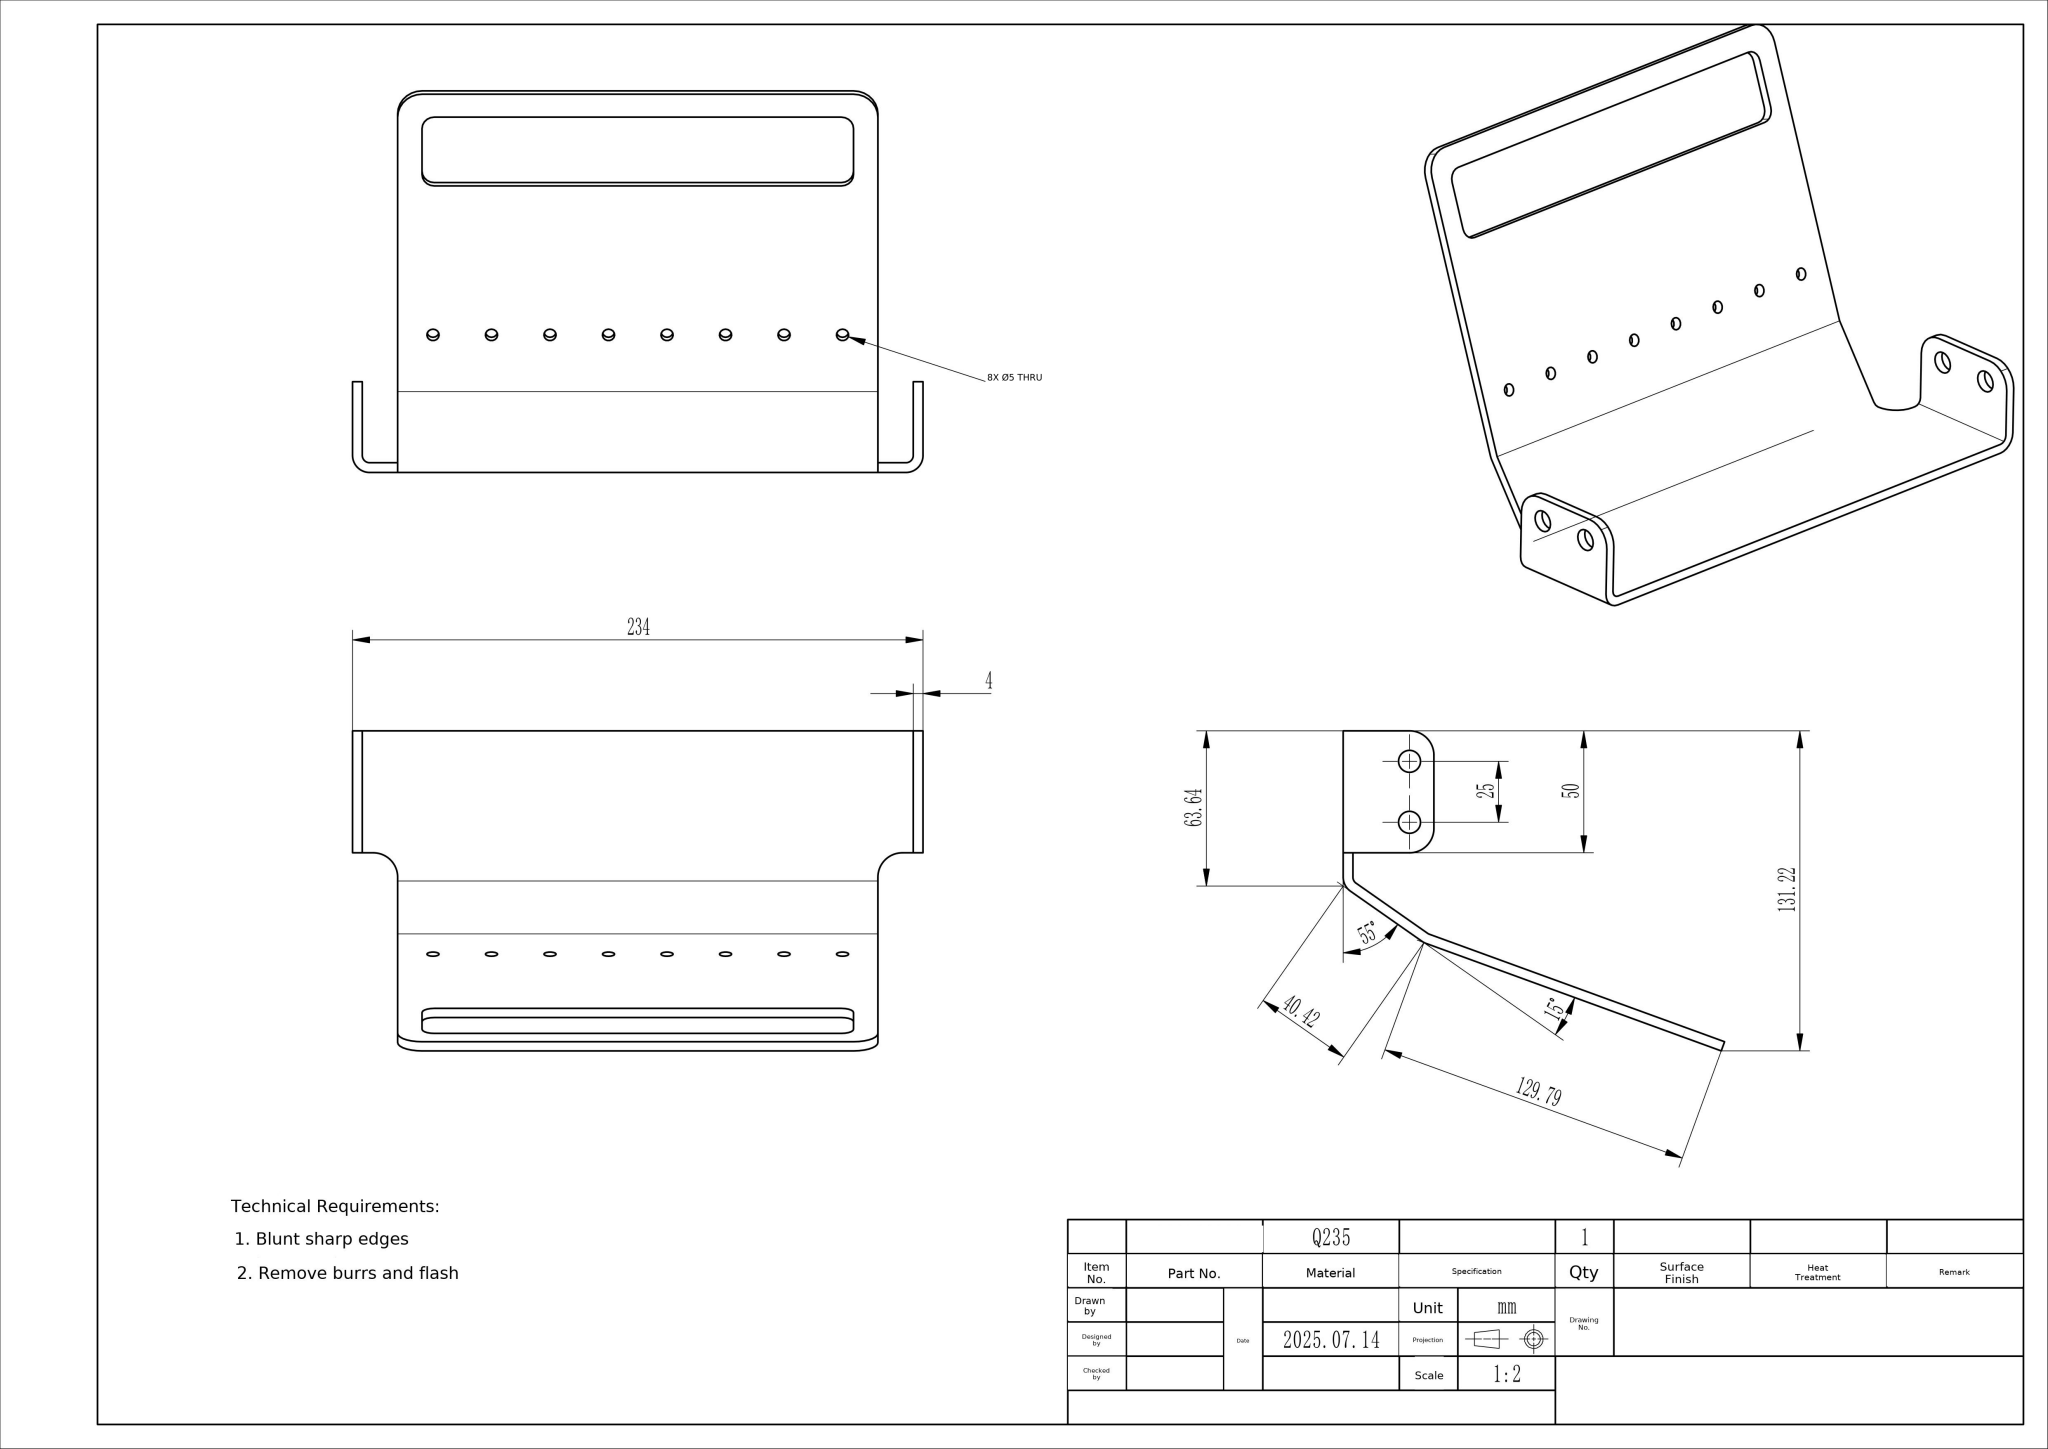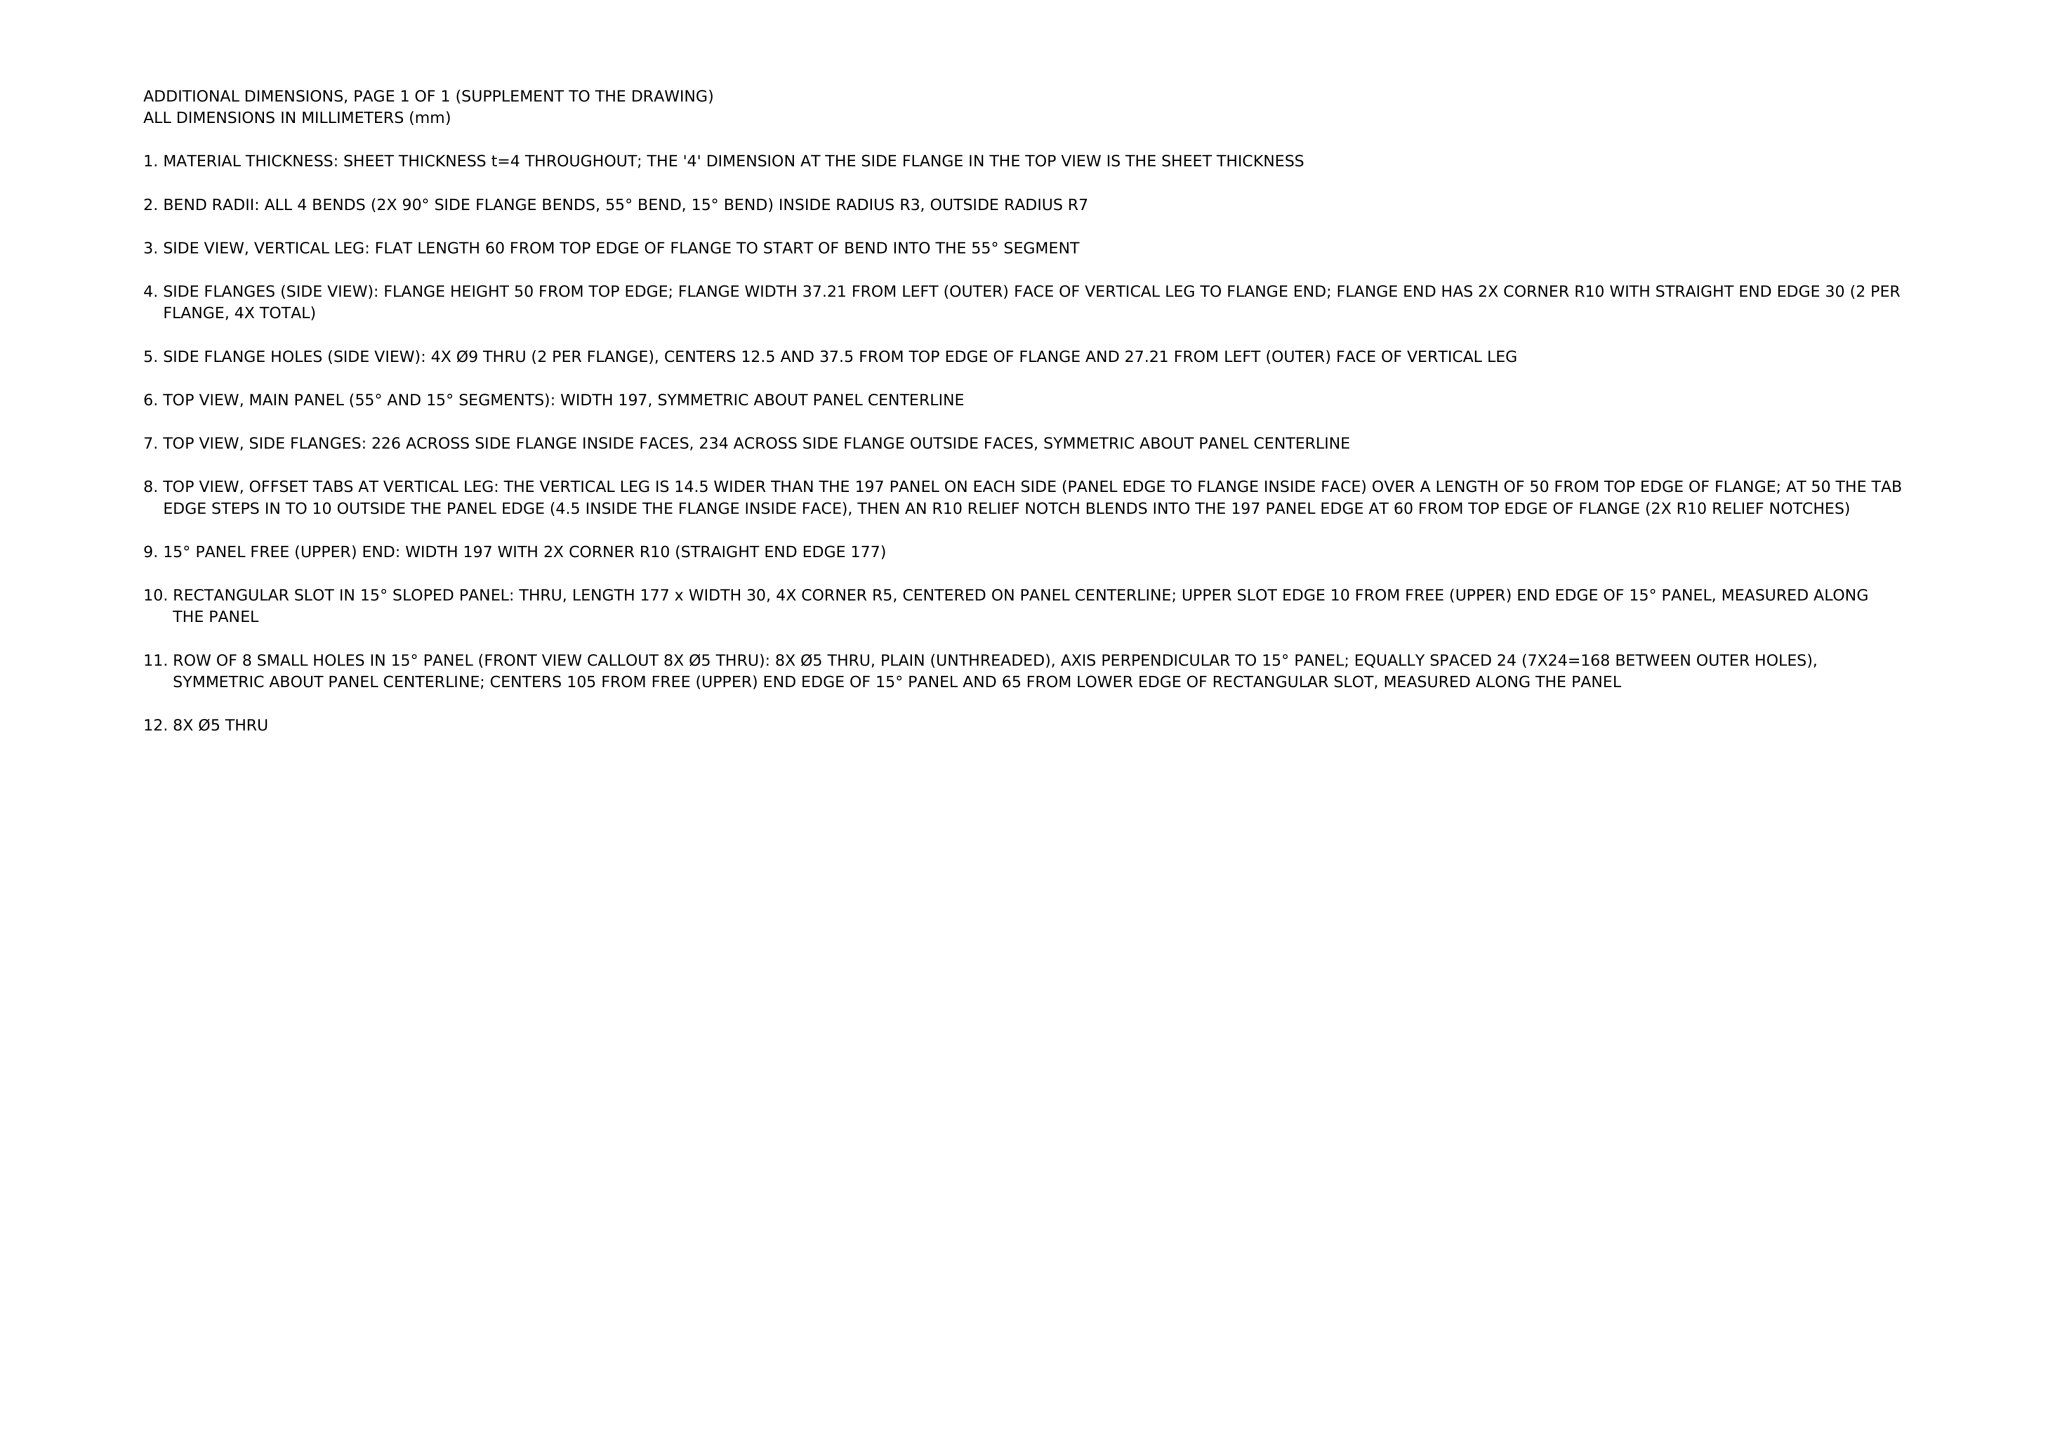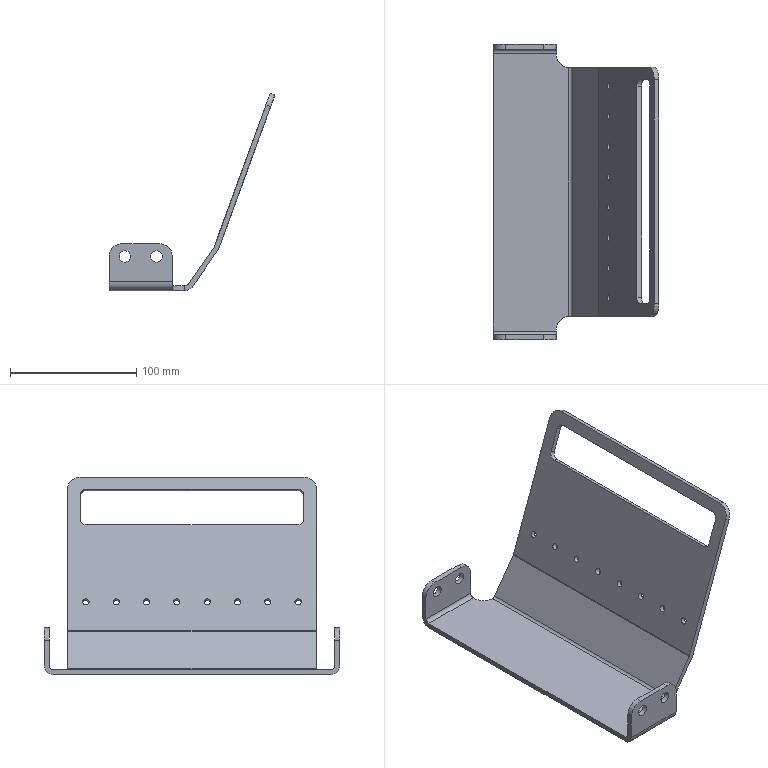Part | NX | mm | 1 solid | 54 faces | box 131.22 x 234 x 156.44 mm | volume 178578 mm3 | cylinder 32 | plane 22 | commonest cylinder face diameters 20 x8 5 x8 9 x4 14 x4 6 x4 10 x4